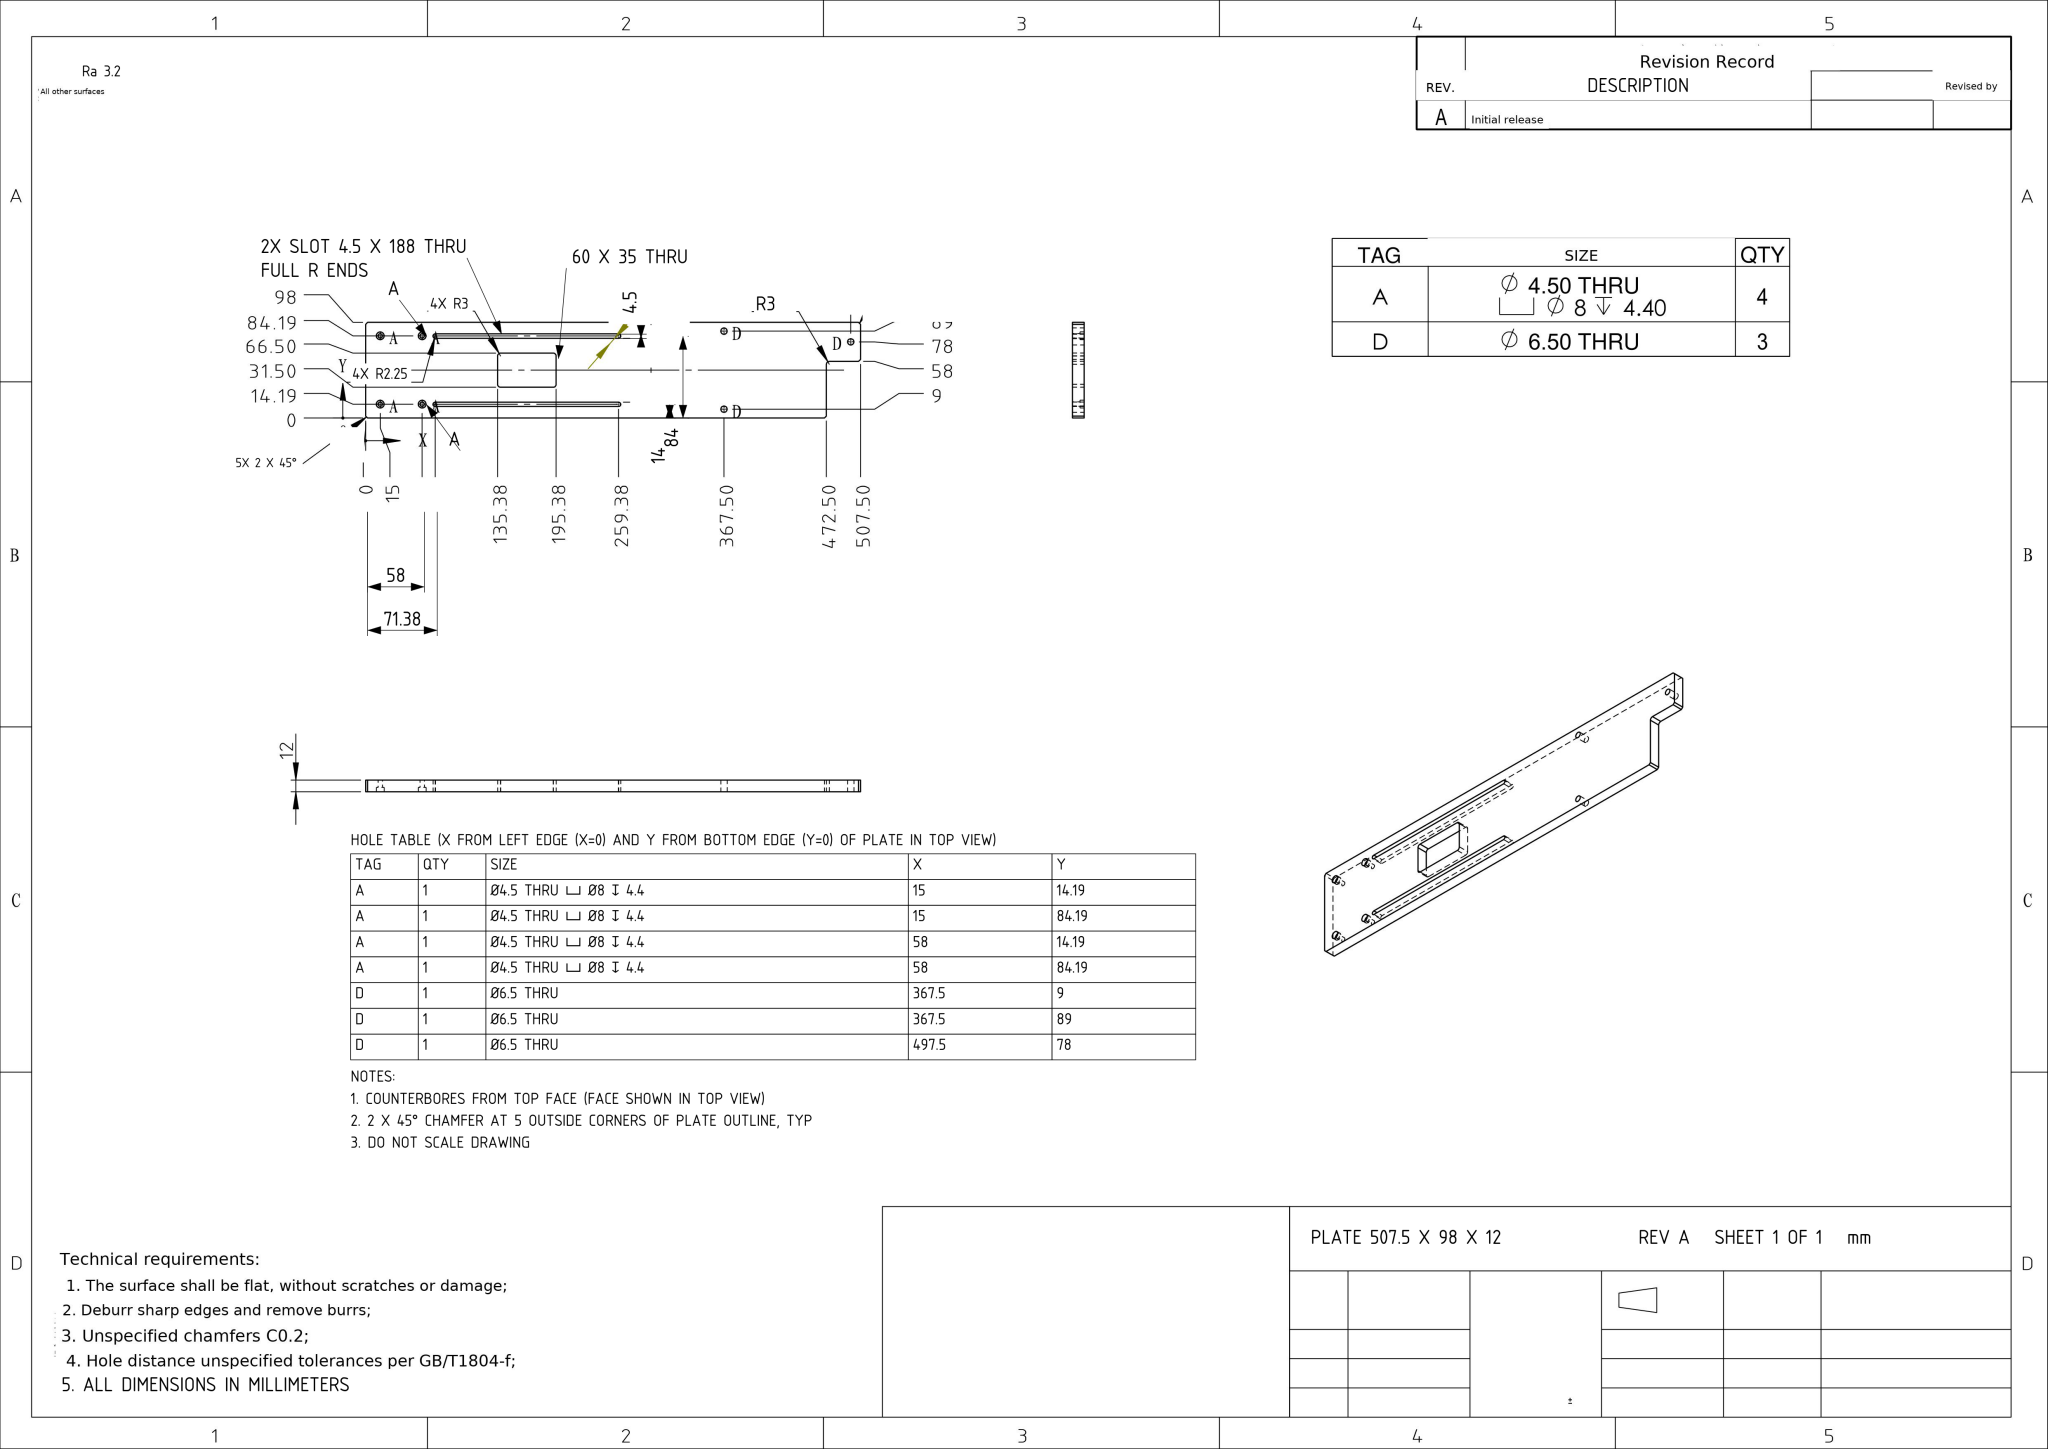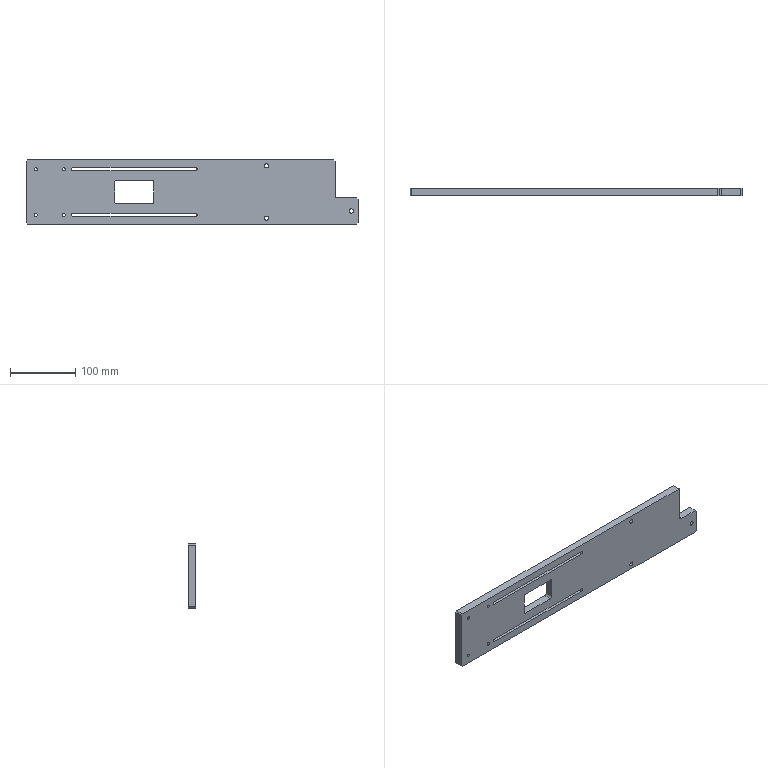Part | NX | mm | 1 solid | 56 faces | box 507.5 x 12 x 98 mm | volume 524007 mm3 | cylinder 31 | plane 25 | commonest cylinder face diameters 4.5 x12 8 x8 6.5 x6 6 x5